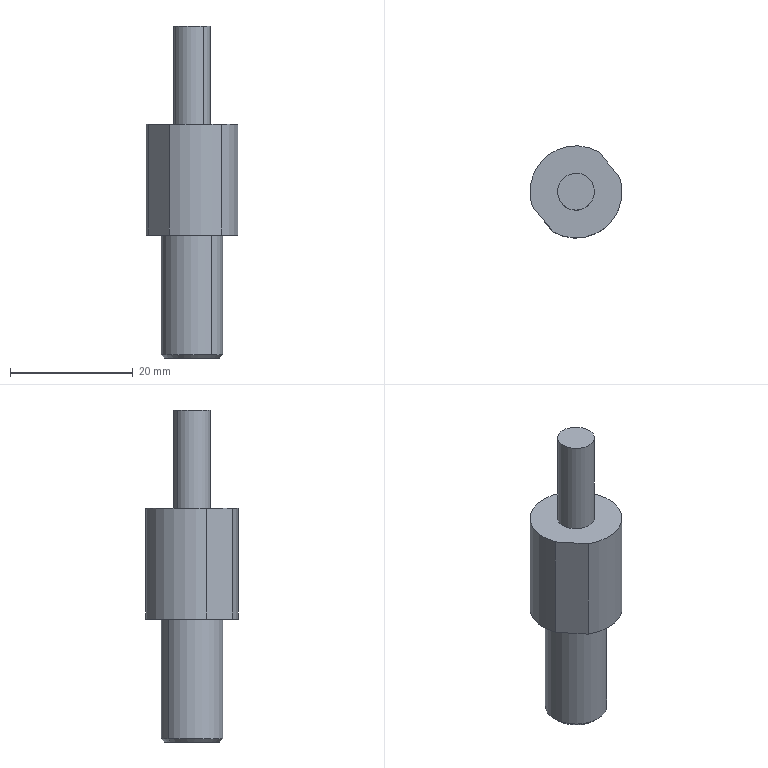Component | SolidWorks | EncoderAxis-1 | 1 solid | 15 faces | box 15 x 15 x 54 mm | volume 5135 mm3 | cylinder 7 | plane 6 | cone 2 | commonest cylinder face diameters 15 x3 6 x2 10 x2
build123d program:
from build123d import *

# Parameters (mm, degrees)
CHAMFER1_SIZE      = 0.5
SKETCH2_W          = 24.567
SKETCH2_H          = 7.758
SKETCH2_W_2        = 25.214
SKETCH2_H_2        = 7.065
CUT_EXTRUDE1_DEPTH = 18


with BuildPart() as part:
    # Sketch1 → Revolve1 (revolve)
    with BuildSketch(Plane.XY, mode=Mode.PRIVATE) as revolve1_sk:
        Polygon((0, 0), (0, 5), (-20, 5), (-20, 7.5), (-38, 7.5), (-38, 3), (-54, 3), (-54, 0), align=None)
    revolve(revolve1_sk.sketch.rotate(Axis((-198.656, 0, 0), (1, 0, 0)), 90), axis=Axis((-198.656, 0, 0), (1, 0, 0)))

    # Chamfer1
    chamfer1_edges = [part.edges().sort_by_distance(p)[0] for p in [
        (0, 0, -5),
    ]]
    chamfer(chamfer1_edges, length=CHAMFER1_SIZE)

    # Sketch2 → Cut-Extrude1 (cut)
    with BuildSketch(Plane.ZY.offset(38)):
        with Locations((0.7254, 10.879)):
            Rectangle(SKETCH2_W, SKETCH2_H)
        with Locations((-0.3829, -10.533)):
            Rectangle(SKETCH2_W_2, SKETCH2_H_2)
    extrude(amount=-CUT_EXTRUDE1_DEPTH, mode=Mode.SUBTRACT)


solid = part.part

# Placed as in the assembly
solid = solid.moved(Location((-299.507, -197.911, 616), (90, 39.46, -90)))
STEP:
#1=COLOUR_RGB('',0.7922,0.8196,0.9333);
#2=FILL_AREA_STYLE_COLOUR('',#1);
#3=FILL_AREA_STYLE('',(#2));
#4=SURFACE_STYLE_FILL_AREA(#3);
#5=SURFACE_SIDE_STYLE('',(#4));
#6=SURFACE_STYLE_USAGE(.BOTH.,#5);
#7=PRESENTATION_STYLE_ASSIGNMENT((#6));
#8=CARTESIAN_POINT('',(-11.904,-7.655,24.252));
#9=VERTEX_POINT('',#8);
#10=CARTESIAN_POINT('',(-11.679,-7.929,24.252));
#11=VERTEX_POINT('',#10);
#12=CARTESIAN_POINT('',(-11.792,-7.792,24.252));
#13=DIRECTION('',(0.,0.,-1.));
#14=DIRECTION('',(0.6355,-0.7721,0.));
#15=AXIS2_PLACEMENT_3D('',#12,#13,#14);
#16=CIRCLE('',#15,0.1772);
#17=EDGE_CURVE('',#9,#11,#16,.T.);
#18=ORIENTED_EDGE('',*,*,#17,.F.);
#19=CARTESIAN_POINT('',(-11.917,-7.64,24.272));
#20=VERTEX_POINT('',#19);
#21=CARTESIAN_POINT('',(-11.917,-7.64,24.272));
#22=DIRECTION('',(-0.4494,0.5459,0.7071));
#23=VECTOR('',#22,39.37);
#24=LINE('',#21,#23);
#25=EDGE_CURVE('',#9,#20,#24,.T.);
#26=ORIENTED_EDGE('',*,*,#25,.T.);
#27=CARTESIAN_POINT('',(-11.666,-7.944,24.272));
#28=VERTEX_POINT('',#27);
#29=CARTESIAN_POINT('',(-11.792,-7.792,24.272));
#30=DIRECTION('',(-0.,-0.,1.));
#31=DIRECTION('',(0.6355,-0.7721,0.));
#32=AXIS2_PLACEMENT_3D('',#29,#30,#31);
#33=CIRCLE('',#32,0.1969);
#34=EDGE_CURVE('',#28,#20,#33,.T.);
#35=ORIENTED_EDGE('',*,*,#34,.F.);
#36=CARTESIAN_POINT('',(-11.666,-7.944,24.272));
#37=DIRECTION('',(0.4494,-0.5459,0.7071));
#38=VECTOR('',#37,39.37);
#39=LINE('',#36,#38);
#40=EDGE_CURVE('',#11,#28,#39,.T.);
#41=ORIENTED_EDGE('',*,*,#40,.F.);
#42=EDGE_LOOP('',(#18,#26,#35,#41));
#43=FACE_OUTER_BOUND('',#42,.T.);
#44=CARTESIAN_POINT('',(-11.792,-7.792,24.272));
#45=DIRECTION('',(-0.,-0.,1.));
#46=DIRECTION('',(0.6355,-0.7721,0.));
#47=AXIS2_PLACEMENT_3D('',#44,#45,#46);
#48=CONICAL_SURFACE('',#47,0.1969,0.7854);
#49=ADVANCED_FACE('',(#43),#48,.T.);
#50=CARTESIAN_POINT('',(-11.717,-7.883,25.748));
#51=VERTEX_POINT('',#50);
#52=CARTESIAN_POINT('',(-11.867,-7.701,25.748));
#53=VERTEX_POINT('',#52);
#54=CARTESIAN_POINT('',(-11.792,-7.792,25.748));
#55=DIRECTION('',(-0.,-0.,1.));
#56=DIRECTION('',(0.6355,-0.7721,0.));
#57=AXIS2_PLACEMENT_3D('',#54,#55,#56);
#58=CIRCLE('',#57,0.1181);
#59=EDGE_CURVE('',#51,#53,#58,.T.);
#60=ORIENTED_EDGE('',*,*,#59,.T.);
#61=CARTESIAN_POINT('',(-11.867,-7.701,26.378));
#62=VERTEX_POINT('',#61);
#63=CARTESIAN_POINT('',(-11.867,-7.701,32.073));
#64=DIRECTION('',(-0.,-0.,1.));
#65=VECTOR('',#64,39.37);
#66=LINE('',#63,#65);
#67=EDGE_CURVE('',#53,#62,#66,.T.);
#68=ORIENTED_EDGE('',*,*,#67,.T.);
#69=CARTESIAN_POINT('',(-11.717,-7.883,26.378));
#70=VERTEX_POINT('',#69);
#71=CARTESIAN_POINT('',(-11.792,-7.792,26.378));
#72=DIRECTION('',(-0.,-0.,1.));
#73=DIRECTION('',(0.6355,-0.7721,0.));
#74=AXIS2_PLACEMENT_3D('',#71,#72,#73);
#75=CIRCLE('',#74,0.1181);
#76=EDGE_CURVE('',#70,#62,#75,.T.);
#77=ORIENTED_EDGE('',*,*,#76,.F.);
#78=CARTESIAN_POINT('',(-11.717,-7.883,32.073));
#79=DIRECTION('',(-0.,-0.,1.));
#80=VECTOR('',#79,39.37);
#81=LINE('',#78,#80);
#82=EDGE_CURVE('',#51,#70,#81,.T.);
#83=ORIENTED_EDGE('',*,*,#82,.F.);
#84=EDGE_LOOP('',(#60,#68,#77,#83));
#85=FACE_OUTER_BOUND('',#84,.T.);
#86=CARTESIAN_POINT('',(-11.792,-7.792,32.073));
#87=DIRECTION('',(-0.,-0.,1.));
#88=DIRECTION('',(0.6355,-0.7721,0.));
#89=AXIS2_PLACEMENT_3D('',#86,#87,#88);
#90=CYLINDRICAL_SURFACE('',#89,0.1181);
#91=ADVANCED_FACE('',(#85),#90,.T.);
#92=CARTESIAN_POINT('',(-11.937,-8.049,25.039));
#93=VERTEX_POINT('',#92);
#94=CARTESIAN_POINT('',(-11.604,-8.02,25.039));
#95=VERTEX_POINT('',#94);
#96=CARTESIAN_POINT('',(-11.792,-7.792,25.039));
#97=DIRECTION('',(-0.,-0.,1.));
#98=DIRECTION('',(0.6355,-0.7721,0.));
#99=AXIS2_PLACEMENT_3D('',#96,#97,#98);
#100=CIRCLE('',#99,0.2953);
#101=EDGE_CURVE('',#93,#95,#100,.T.);
#102=ORIENTED_EDGE('',*,*,#101,.T.);
#103=CARTESIAN_POINT('',(-11.604,-8.02,25.748));
#104=VERTEX_POINT('',#103);
#105=CARTESIAN_POINT('',(-11.604,-8.02,32.073));
#106=DIRECTION('',(-0.,-0.,1.));
#107=VECTOR('',#106,39.37);
#108=LINE('',#105,#107);
#109=EDGE_CURVE('',#95,#104,#108,.T.);
#110=ORIENTED_EDGE('',*,*,#109,.T.);
#111=CARTESIAN_POINT('',(-11.937,-8.049,25.748));
#112=VERTEX_POINT('',#111);
#113=CARTESIAN_POINT('',(-11.792,-7.792,25.748));
#114=DIRECTION('',(-0.,-0.,1.));
#115=DIRECTION('',(0.6355,-0.7721,0.));
#116=AXIS2_PLACEMENT_3D('',#113,#114,#115);
#117=CIRCLE('',#116,0.2953);
#118=EDGE_CURVE('',#112,#104,#117,.T.);
#119=ORIENTED_EDGE('',*,*,#118,.F.);
#120=CARTESIAN_POINT('',(-11.937,-8.049,32.073));
#121=DIRECTION('',(0.,0.,-1.));
#122=VECTOR('',#121,39.37);
#123=LINE('',#120,#122);
#124=EDGE_CURVE('',#112,#93,#123,.T.);
#125=ORIENTED_EDGE('',*,*,#124,.T.);
#126=EDGE_LOOP('',(#102,#110,#119,#125));
#127=FACE_OUTER_BOUND('',#126,.T.);
#128=CARTESIAN_POINT('',(-11.792,-7.792,32.073));
#129=DIRECTION('',(-0.,-0.,1.));
#130=DIRECTION('',(0.6355,-0.7721,0.));
#131=AXIS2_PLACEMENT_3D('',#128,#129,#130);
#132=CYLINDRICAL_SURFACE('',#131,0.2953);
#133=ADVANCED_FACE('',(#127),#132,.T.);
#134=ORIENTED_EDGE('',*,*,#34,.T.);
#135=CARTESIAN_POINT('',(-11.917,-7.64,25.039));
#136=VERTEX_POINT('',#135);
#137=CARTESIAN_POINT('',(-11.917,-7.64,32.073));
#138=DIRECTION('',(-0.,-0.,1.));
#139=VECTOR('',#138,39.37);
#140=LINE('',#137,#139);
#141=EDGE_CURVE('',#20,#136,#140,.T.);
#142=ORIENTED_EDGE('',*,*,#141,.T.);
#143=CARTESIAN_POINT('',(-11.666,-7.944,25.039));
#144=VERTEX_POINT('',#143);
#145=CARTESIAN_POINT('',(-11.792,-7.792,25.039));
#146=DIRECTION('',(-0.,-0.,1.));
#147=DIRECTION('',(0.6355,-0.7721,0.));
#148=AXIS2_PLACEMENT_3D('',#145,#146,#147);
#149=CIRCLE('',#148,0.1969);
#150=EDGE_CURVE('',#144,#136,#149,.T.);
#151=ORIENTED_EDGE('',*,*,#150,.F.);
#152=CARTESIAN_POINT('',(-11.666,-7.944,32.073));
#153=DIRECTION('',(-0.,-0.,1.));
#154=VECTOR('',#153,39.37);
#155=LINE('',#152,#154);
#156=EDGE_CURVE('',#28,#144,#155,.T.);
#157=ORIENTED_EDGE('',*,*,#156,.F.);
#158=EDGE_LOOP('',(#134,#142,#151,#157));
#159=FACE_OUTER_BOUND('',#158,.T.);
#160=CARTESIAN_POINT('',(-11.792,-7.792,32.073));
#161=DIRECTION('',(-0.,-0.,1.));
#162=DIRECTION('',(0.6355,-0.7721,0.));
#163=AXIS2_PLACEMENT_3D('',#160,#161,#162);
#164=CYLINDRICAL_SURFACE('',#163,0.1969);
#165=ADVANCED_FACE('',(#159),#164,.T.);
#166=CARTESIAN_POINT('',(-11.646,-7.535,25.039));
#167=VERTEX_POINT('',#166);
#168=CARTESIAN_POINT('',(-12.072,-7.885,25.039));
#169=VERTEX_POINT('',#168);
#170=CARTESIAN_POINT('',(-11.792,-7.792,25.039));
#171=DIRECTION('',(-0.,-0.,1.));
#172=DIRECTION('',(0.6355,-0.7721,0.));
#173=AXIS2_PLACEMENT_3D('',#170,#171,#172);
#174=CIRCLE('',#173,0.2953);
#175=EDGE_CURVE('',#167,#169,#174,.T.);
#176=ORIENTED_EDGE('',*,*,#175,.T.);
#177=CARTESIAN_POINT('',(-12.072,-7.885,25.748));
#178=VERTEX_POINT('',#177);
#179=CARTESIAN_POINT('',(-12.072,-7.885,32.073));
#180=DIRECTION('',(-0.,-0.,1.));
#181=VECTOR('',#180,39.37);
#182=LINE('',#179,#181);
#183=EDGE_CURVE('',#169,#178,#182,.T.);
#184=ORIENTED_EDGE('',*,*,#183,.T.);
#185=CARTESIAN_POINT('',(-11.646,-7.535,25.748));
#186=VERTEX_POINT('',#185);
#187=CARTESIAN_POINT('',(-11.792,-7.792,25.748));
#188=DIRECTION('',(-0.,-0.,1.));
#189=DIRECTION('',(0.6355,-0.7721,0.));
#190=AXIS2_PLACEMENT_3D('',#187,#188,#189);
#191=CIRCLE('',#190,0.2953);
#192=EDGE_CURVE('',#186,#178,#191,.T.);
#193=ORIENTED_EDGE('',*,*,#192,.F.);
#194=CARTESIAN_POINT('',(-11.646,-7.535,32.073));
#195=DIRECTION('',(0.,0.,-1.));
#196=VECTOR('',#195,39.37);
#197=LINE('',#194,#196);
#198=EDGE_CURVE('',#186,#167,#197,.T.);
#199=ORIENTED_EDGE('',*,*,#198,.T.);
#200=EDGE_LOOP('',(#176,#184,#193,#199));
#201=FACE_OUTER_BOUND('',#200,.T.);
#202=CARTESIAN_POINT('',(-11.792,-7.792,32.073));
#203=DIRECTION('',(-0.,-0.,1.));
#204=DIRECTION('',(0.6355,-0.7721,0.));
#205=AXIS2_PLACEMENT_3D('',#202,#203,#204);
#206=CYLINDRICAL_SURFACE('',#205,0.2953);
#207=ADVANCED_FACE('',(#201),#206,.T.);
#208=CARTESIAN_POINT('',(-11.792,-7.792,24.252));
#209=DIRECTION('',(0.,0.,-1.));
#210=DIRECTION('',(0.6355,-0.7721,0.));
#211=AXIS2_PLACEMENT_3D('',#208,#209,#210);
#212=CIRCLE('',#211,0.1772);
#213=EDGE_CURVE('',#11,#9,#212,.T.);
#214=ORIENTED_EDGE('',*,*,#213,.T.);
#215=ORIENTED_EDGE('',*,*,#17,.T.);
#216=EDGE_LOOP('',(#214,#215));
#217=FACE_OUTER_BOUND('',#216,.T.);
#218=CARTESIAN_POINT('',(-11.792,-7.792,24.252));
#219=DIRECTION('',(-0.,-0.,1.));
#220=DIRECTION('',(0.6355,-0.7721,-0.));
#221=AXIS2_PLACEMENT_3D('',#218,#219,#220);
#222=PLANE('',#221);
#223=ADVANCED_FACE('',(#217),#222,.F.);
#224=ORIENTED_EDGE('',*,*,#141,.F.);
#225=CARTESIAN_POINT('',(-11.792,-7.792,24.272));
#226=DIRECTION('',(-0.,-0.,1.));
#227=DIRECTION('',(0.6355,-0.7721,0.));
#228=AXIS2_PLACEMENT_3D('',#225,#226,#227);
#229=CIRCLE('',#228,0.1969);
#230=EDGE_CURVE('',#20,#28,#229,.T.);
#231=ORIENTED_EDGE('',*,*,#230,.T.);
#232=ORIENTED_EDGE('',*,*,#156,.T.);
#233=CARTESIAN_POINT('',(-11.792,-7.792,25.039));
#234=DIRECTION('',(-0.,-0.,1.));
#235=DIRECTION('',(0.6355,-0.7721,0.));
#236=AXIS2_PLACEMENT_3D('',#233,#234,#235);
#237=CIRCLE('',#236,0.1969);
#238=EDGE_CURVE('',#136,#144,#237,.T.);
#239=ORIENTED_EDGE('',*,*,#238,.F.);
#240=EDGE_LOOP('',(#224,#231,#232,#239));
#241=FACE_OUTER_BOUND('',#240,.T.);
#242=CARTESIAN_POINT('',(-11.792,-7.792,32.073));
#243=DIRECTION('',(-0.,-0.,1.));
#244=DIRECTION('',(0.6355,-0.7721,0.));
#245=AXIS2_PLACEMENT_3D('',#242,#243,#244);
#246=CYLINDRICAL_SURFACE('',#245,0.1969);
#247=ADVANCED_FACE('',(#241),#246,.T.);
#248=ORIENTED_EDGE('',*,*,#101,.F.);
#249=CARTESIAN_POINT('',(-11.699,-8.338,25.039));
#250=DIRECTION('',(-0.6355,0.7721,0.));
#251=VECTOR('',#250,39.37);
#252=LINE('',#249,#251);
#253=EDGE_CURVE('',#93,#169,#252,.T.);
#254=ORIENTED_EDGE('',*,*,#253,.T.);
#255=ORIENTED_EDGE('',*,*,#175,.F.);
#256=CARTESIAN_POINT('',(-11.511,-7.698,25.039));
#257=VERTEX_POINT('',#256);
#258=CARTESIAN_POINT('',(-11.868,-7.265,25.039));
#259=DIRECTION('',(0.6355,-0.7721,-0.));
#260=VECTOR('',#259,39.37);
#261=LINE('',#258,#260);
#262=EDGE_CURVE('',#167,#257,#261,.T.);
#263=ORIENTED_EDGE('',*,*,#262,.T.);
#264=CARTESIAN_POINT('',(-11.792,-7.792,25.039));
#265=DIRECTION('',(-0.,-0.,1.));
#266=DIRECTION('',(0.6355,-0.7721,0.));
#267=AXIS2_PLACEMENT_3D('',#264,#265,#266);
#268=CIRCLE('',#267,0.2953);
#269=EDGE_CURVE('',#95,#257,#268,.T.);
#270=ORIENTED_EDGE('',*,*,#269,.F.);
#271=EDGE_LOOP('',(#248,#254,#255,#263,#270));
#272=FACE_OUTER_BOUND('',#271,.T.);
#273=ORIENTED_EDGE('',*,*,#150,.T.);
#274=ORIENTED_EDGE('',*,*,#238,.T.);
#275=EDGE_LOOP('',(#273,#274));
#276=FACE_BOUND('',#275,.T.);
#277=CARTESIAN_POINT('',(-11.64,-7.667,25.039));
#278=DIRECTION('',(-0.,-0.,1.));
#279=DIRECTION('',(0.6355,-0.7721,-0.));
#280=AXIS2_PLACEMENT_3D('',#277,#278,#279);
#281=PLANE('',#280);
#282=ADVANCED_FACE('',(#272,#276),#281,.F.);
#283=ORIENTED_EDGE('',*,*,#109,.F.);
#284=ORIENTED_EDGE('',*,*,#269,.T.);
#285=CARTESIAN_POINT('',(-11.511,-7.698,25.748));
#286=VERTEX_POINT('',#285);
#287=CARTESIAN_POINT('',(-11.511,-7.698,32.073));
#288=DIRECTION('',(-0.,-0.,1.));
#289=VECTOR('',#288,39.37);
#290=LINE('',#287,#289);
#291=EDGE_CURVE('',#257,#286,#290,.T.);
#292=ORIENTED_EDGE('',*,*,#291,.T.);
#293=CARTESIAN_POINT('',(-11.792,-7.792,25.748));
#294=DIRECTION('',(-0.,-0.,1.));
#295=DIRECTION('',(0.6355,-0.7721,0.));
#296=AXIS2_PLACEMENT_3D('',#293,#294,#295);
#297=CIRCLE('',#296,0.2953);
#298=EDGE_CURVE('',#104,#286,#297,.T.);
#299=ORIENTED_EDGE('',*,*,#298,.F.);
#300=EDGE_LOOP('',(#283,#284,#292,#299));
#301=FACE_OUTER_BOUND('',#300,.T.);
#302=CARTESIAN_POINT('',(-11.792,-7.792,32.073));
#303=DIRECTION('',(-0.,-0.,1.));
#304=DIRECTION('',(0.6355,-0.7721,0.));
#305=AXIS2_PLACEMENT_3D('',#302,#303,#304);
#306=CYLINDRICAL_SURFACE('',#305,0.2953);
#307=ADVANCED_FACE('',(#301),#306,.T.);
#308=ORIENTED_EDGE('',*,*,#59,.F.);
#309=CARTESIAN_POINT('',(-11.792,-7.792,25.748));
#310=DIRECTION('',(-0.,-0.,1.));
#311=DIRECTION('',(0.6355,-0.7721,0.));
#312=AXIS2_PLACEMENT_3D('',#309,#310,#311);
#313=CIRCLE('',#312,0.1181);
#314=EDGE_CURVE('',#53,#51,#313,.T.);
#315=ORIENTED_EDGE('',*,*,#314,.F.);
#316=EDGE_LOOP('',(#308,#315));
#317=FACE_BOUND('',#316,.T.);
#318=ORIENTED_EDGE('',*,*,#192,.T.);
#319=CARTESIAN_POINT('',(-12.004,-7.967,25.748));
#320=DIRECTION('',(0.6355,-0.7721,-0.));
#321=VECTOR('',#320,39.37);
#322=LINE('',#319,#321);
#323=EDGE_CURVE('',#178,#112,#322,.T.);
#324=ORIENTED_EDGE('',*,*,#323,.T.);
#325=ORIENTED_EDGE('',*,*,#118,.T.);
#326=ORIENTED_EDGE('',*,*,#298,.T.);
#327=CARTESIAN_POINT('',(-11.579,-7.617,25.748));
#328=DIRECTION('',(-0.6355,0.7721,0.));
#329=VECTOR('',#328,39.37);
#330=LINE('',#327,#329);
#331=EDGE_CURVE('',#286,#186,#330,.T.);
#332=ORIENTED_EDGE('',*,*,#331,.T.);
#333=EDGE_LOOP('',(#318,#324,#325,#326,#332));
#334=FACE_OUTER_BOUND('',#333,.T.);
#335=CARTESIAN_POINT('',(-11.564,-7.604,25.748));
#336=DIRECTION('',(0.,0.,-1.));
#337=DIRECTION('',(-0.6355,0.7721,0.));
#338=AXIS2_PLACEMENT_3D('',#335,#336,#337);
#339=PLANE('',#338);
#340=ADVANCED_FACE('',(#317,#334),#339,.F.);
#341=ORIENTED_EDGE('',*,*,#67,.F.);
#342=ORIENTED_EDGE('',*,*,#314,.T.);
#343=ORIENTED_EDGE('',*,*,#82,.T.);
#344=CARTESIAN_POINT('',(-11.792,-7.792,26.378));
#345=DIRECTION('',(-0.,-0.,1.));
#346=DIRECTION('',(0.6355,-0.7721,0.));
#347=AXIS2_PLACEMENT_3D('',#344,#345,#346);
#348=CIRCLE('',#347,0.1181);
#349=EDGE_CURVE('',#62,#70,#348,.T.);
#350=ORIENTED_EDGE('',*,*,#349,.F.);
#351=EDGE_LOOP('',(#341,#342,#343,#350));
#352=FACE_OUTER_BOUND('',#351,.T.);
#353=CARTESIAN_POINT('',(-11.792,-7.792,32.073));
#354=DIRECTION('',(-0.,-0.,1.));
#355=DIRECTION('',(0.6355,-0.7721,0.));
#356=AXIS2_PLACEMENT_3D('',#353,#354,#355);
#357=CYLINDRICAL_SURFACE('',#356,0.1181);
#358=ADVANCED_FACE('',(#352),#357,.T.);
#359=ORIENTED_EDGE('',*,*,#76,.T.);
#360=ORIENTED_EDGE('',*,*,#349,.T.);
#361=EDGE_LOOP('',(#359,#360));
#362=FACE_OUTER_BOUND('',#361,.T.);
#363=CARTESIAN_POINT('',(-11.7,-7.717,26.378));
#364=DIRECTION('',(0.,0.,-1.));
#365=DIRECTION('',(-0.6355,0.7721,0.));
#366=AXIS2_PLACEMENT_3D('',#363,#364,#365);
#367=PLANE('',#366);
#368=ADVANCED_FACE('',(#362),#367,.F.);
#369=ORIENTED_EDGE('',*,*,#25,.F.);
#370=ORIENTED_EDGE('',*,*,#213,.F.);
#371=ORIENTED_EDGE('',*,*,#40,.T.);
#372=ORIENTED_EDGE('',*,*,#230,.F.);
#373=EDGE_LOOP('',(#369,#370,#371,#372));
#374=FACE_OUTER_BOUND('',#373,.T.);
#375=CARTESIAN_POINT('',(-11.792,-7.792,24.272));
#376=DIRECTION('',(-0.,-0.,1.));
#377=DIRECTION('',(0.6355,-0.7721,0.));
#378=AXIS2_PLACEMENT_3D('',#375,#376,#377);
#379=CONICAL_SURFACE('',#378,0.1969,0.7854);
#380=ADVANCED_FACE('',(#374),#379,.T.);
#381=ORIENTED_EDGE('',*,*,#262,.F.);
#382=ORIENTED_EDGE('',*,*,#198,.F.);
#383=ORIENTED_EDGE('',*,*,#331,.F.);
#384=ORIENTED_EDGE('',*,*,#291,.F.);
#385=EDGE_LOOP('',(#381,#382,#383,#384));
#386=FACE_OUTER_BOUND('',#385,.T.);
#387=CARTESIAN_POINT('',(-11.868,-7.265,25.039));
#388=DIRECTION('',(-0.7721,-0.6355,-0.));
#389=DIRECTION('',(-0.6355,0.7721,0.));
#390=AXIS2_PLACEMENT_3D('',#387,#388,#389);
#391=PLANE('',#390);
#392=ADVANCED_FACE('',(#386),#391,.F.);
#393=ORIENTED_EDGE('',*,*,#253,.F.);
#394=ORIENTED_EDGE('',*,*,#124,.F.);
#395=ORIENTED_EDGE('',*,*,#323,.F.);
#396=ORIENTED_EDGE('',*,*,#183,.F.);
#397=EDGE_LOOP('',(#393,#394,#395,#396));
#398=FACE_OUTER_BOUND('',#397,.T.);
#399=CARTESIAN_POINT('',(-11.699,-8.338,25.039));
#400=DIRECTION('',(0.7721,0.6355,0.));
#401=DIRECTION('',(0.6355,-0.7721,-0.));
#402=AXIS2_PLACEMENT_3D('',#399,#400,#401);
#403=PLANE('',#402);
#404=ADVANCED_FACE('',(#398),#403,.F.);
#405=CLOSED_SHELL('',(#49,#91,#133,#165,#207,#223,#247,#282,#307,#340,#358,#368,#380,#392,#404));
#406=MANIFOLD_SOLID_BREP('',#405);
#407=STYLED_ITEM('',(#7),#406);
#408=(LENGTH_UNIT()NAMED_UNIT(*)SI_UNIT($,.METRE.));
#409=LENGTH_MEASURE_WITH_UNIT(LENGTH_MEASURE(0.0254),#408);
#410=DIMENSIONAL_EXPONENTS(1.,0.,0.,0.,0.,0.,0.);
#411=(CONVERSION_BASED_UNIT('',#409)LENGTH_UNIT()NAMED_UNIT(#410));
#412=UNCERTAINTY_MEASURE_WITH_UNIT(LENGTH_MEASURE(0.00001),#411,'','');
#413=(NAMED_UNIT(*)PLANE_ANGLE_UNIT()SI_UNIT($,.RADIAN.));
#414=(NAMED_UNIT(*)SI_UNIT($,.STERADIAN.)SOLID_ANGLE_UNIT());
#415=(GEOMETRIC_REPRESENTATION_CONTEXT(3)GLOBAL_UNCERTAINTY_ASSIGNED_CONTEXT((#412))GLOBAL_UNIT_ASSIGNED_CONTEXT((#411,#413,#414))REPRESENTATION_CONTEXT('',''));
#416=MECHANICAL_DESIGN_GEOMETRIC_PRESENTATION_REPRESENTATION('',(#407),#415);
#417=CARTESIAN_POINT('',(0.,0.,0.));
#418=DIRECTION('',(0.,0.,1.));
#419=DIRECTION('',(1.,0.,0.));
#420=AXIS2_PLACEMENT_3D('',#417,#418,#419);
#421=(LENGTH_UNIT()NAMED_UNIT(*)SI_UNIT($,.METRE.));
#422=LENGTH_MEASURE_WITH_UNIT(LENGTH_MEASURE(0.0254),#421);
#423=DIMENSIONAL_EXPONENTS(1.,0.,0.,0.,0.,0.,0.);
#424=(CONVERSION_BASED_UNIT('',#422)LENGTH_UNIT()NAMED_UNIT(#423));
#425=UNCERTAINTY_MEASURE_WITH_UNIT(LENGTH_MEASURE(0.00001),#424,'','');
#426=(NAMED_UNIT(*)PLANE_ANGLE_UNIT()SI_UNIT($,.RADIAN.));
#427=(NAMED_UNIT(*)SI_UNIT($,.STERADIAN.)SOLID_ANGLE_UNIT());
#428=(GEOMETRIC_REPRESENTATION_CONTEXT(3)GLOBAL_UNCERTAINTY_ASSIGNED_CONTEXT((#425))GLOBAL_UNIT_ASSIGNED_CONTEXT((#424,#426,#427))REPRESENTATION_CONTEXT('',''));
#429=ADVANCED_BREP_SHAPE_REPRESENTATION('',(#406,#420),#428);
#430=PRESENTATION_LAYER_ASSIGNMENT('','',(#407));